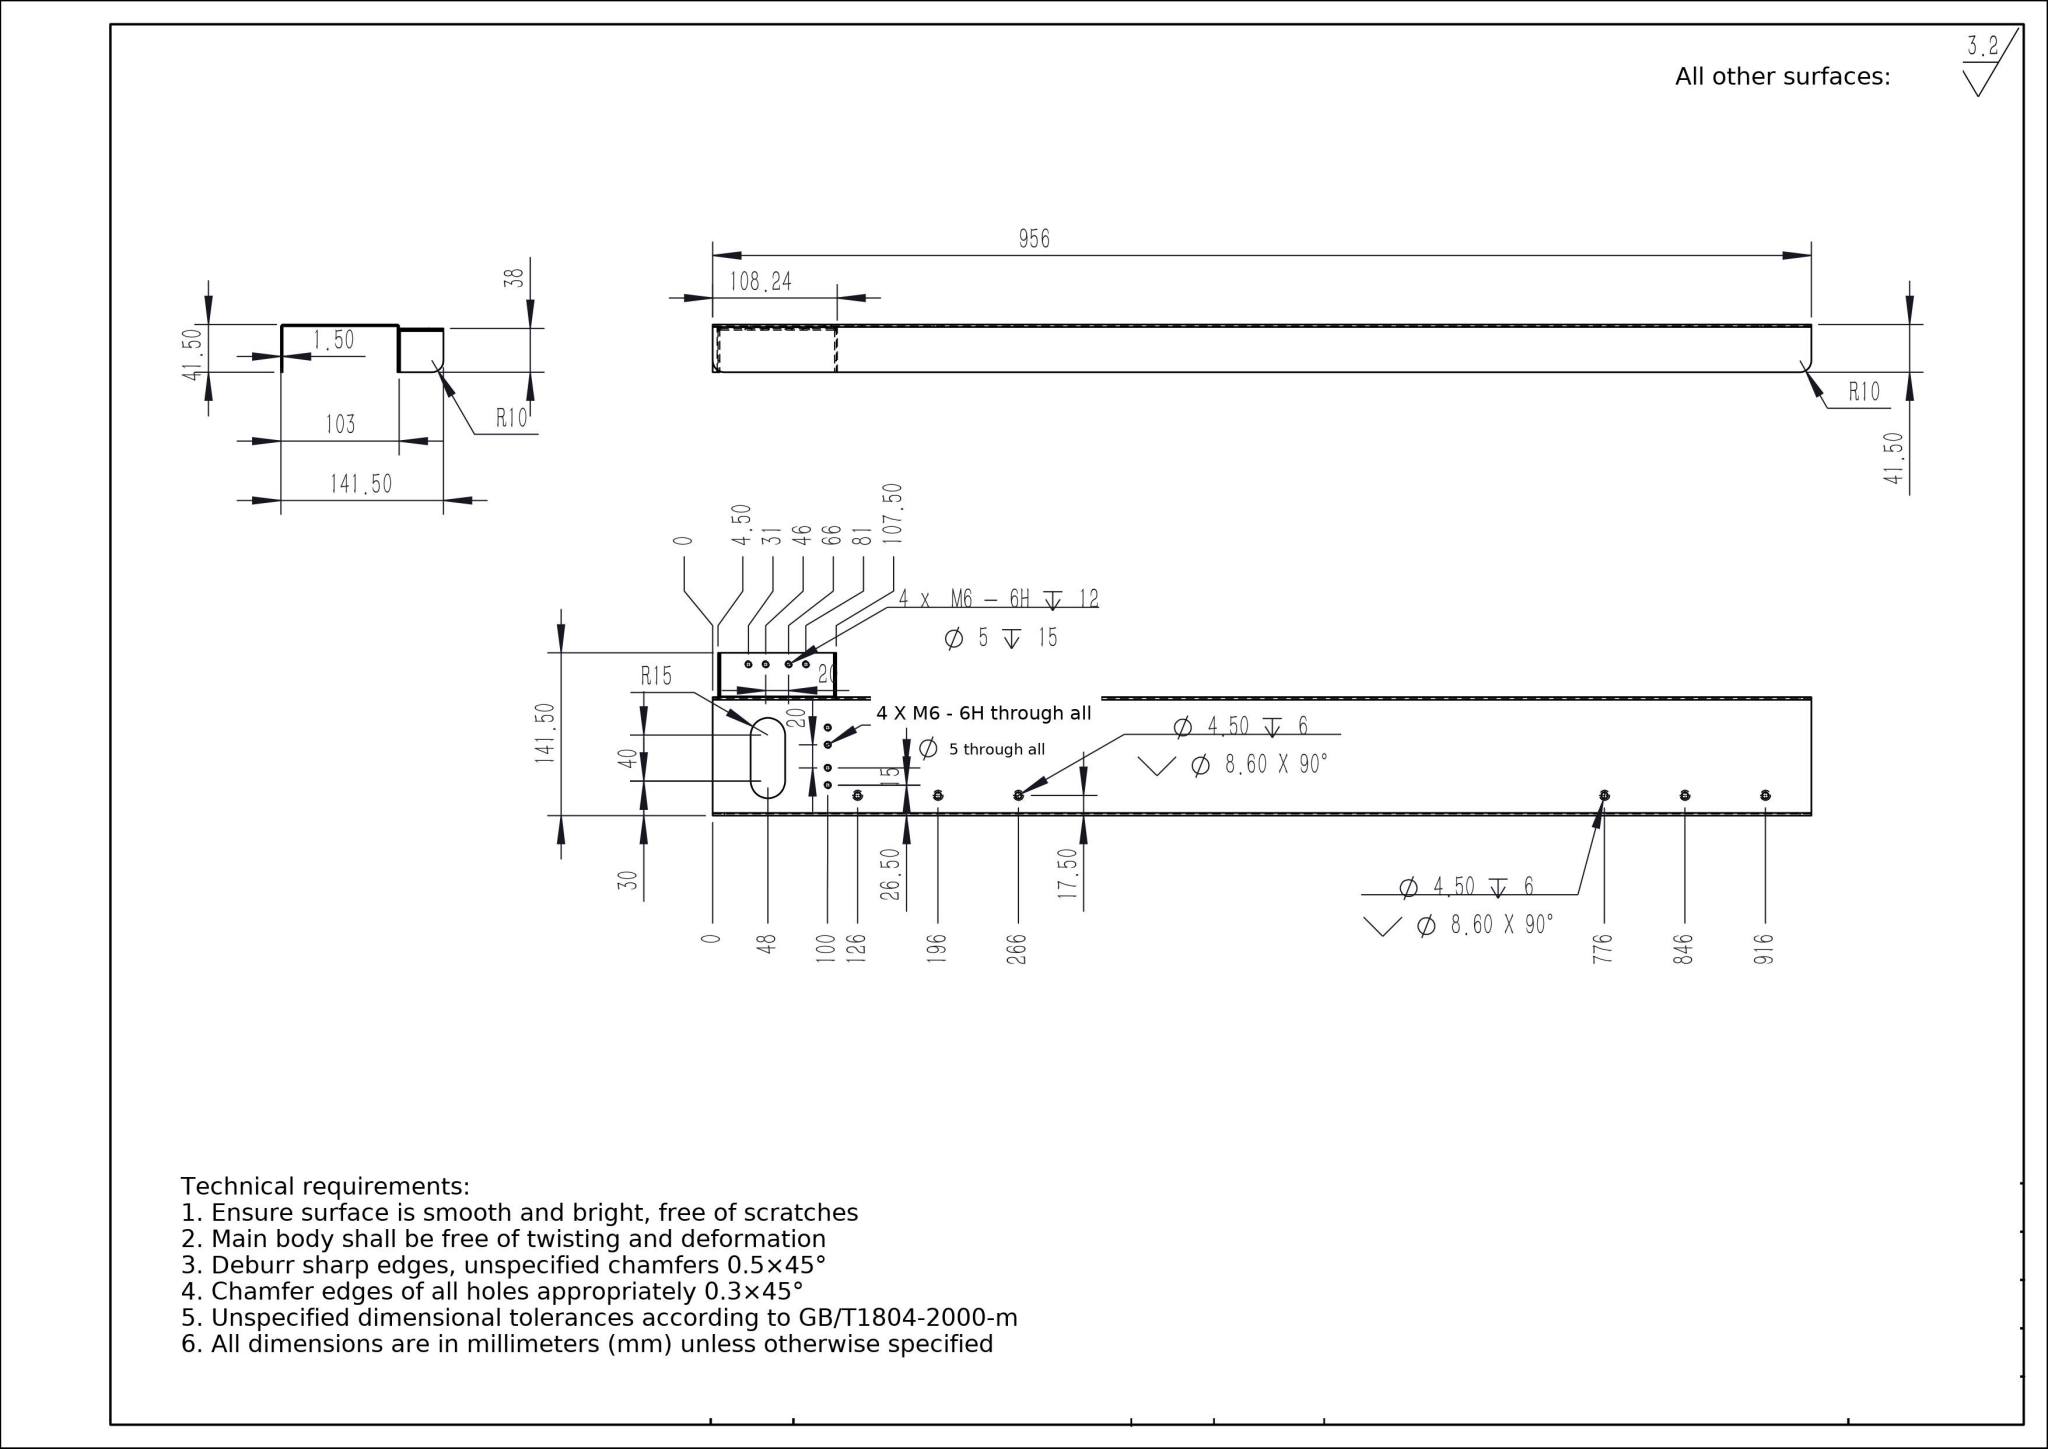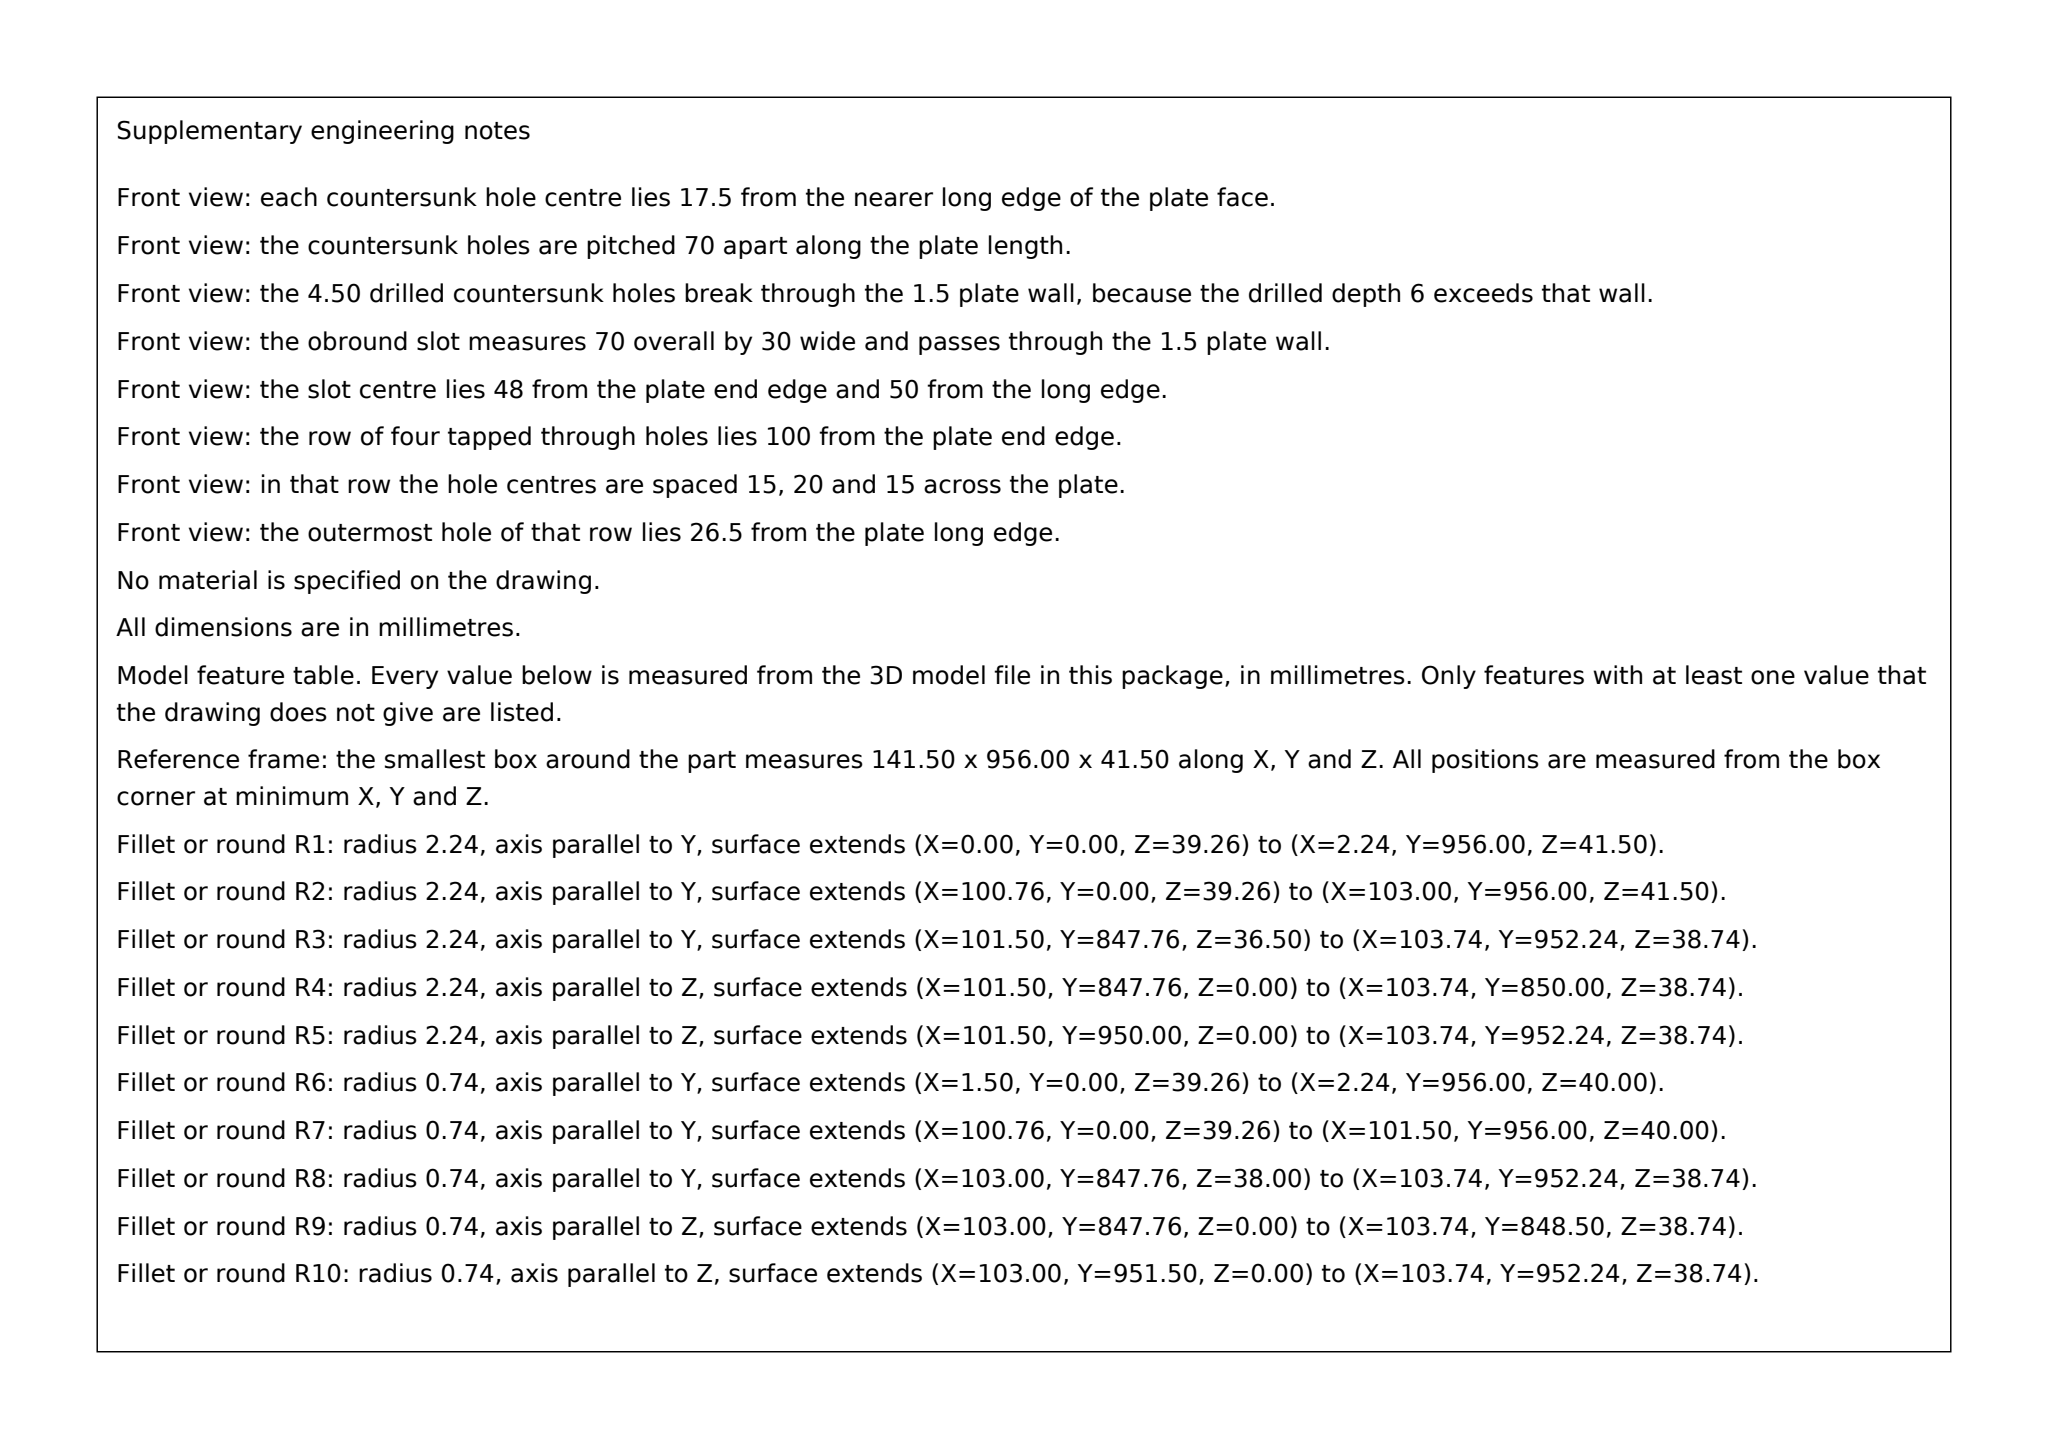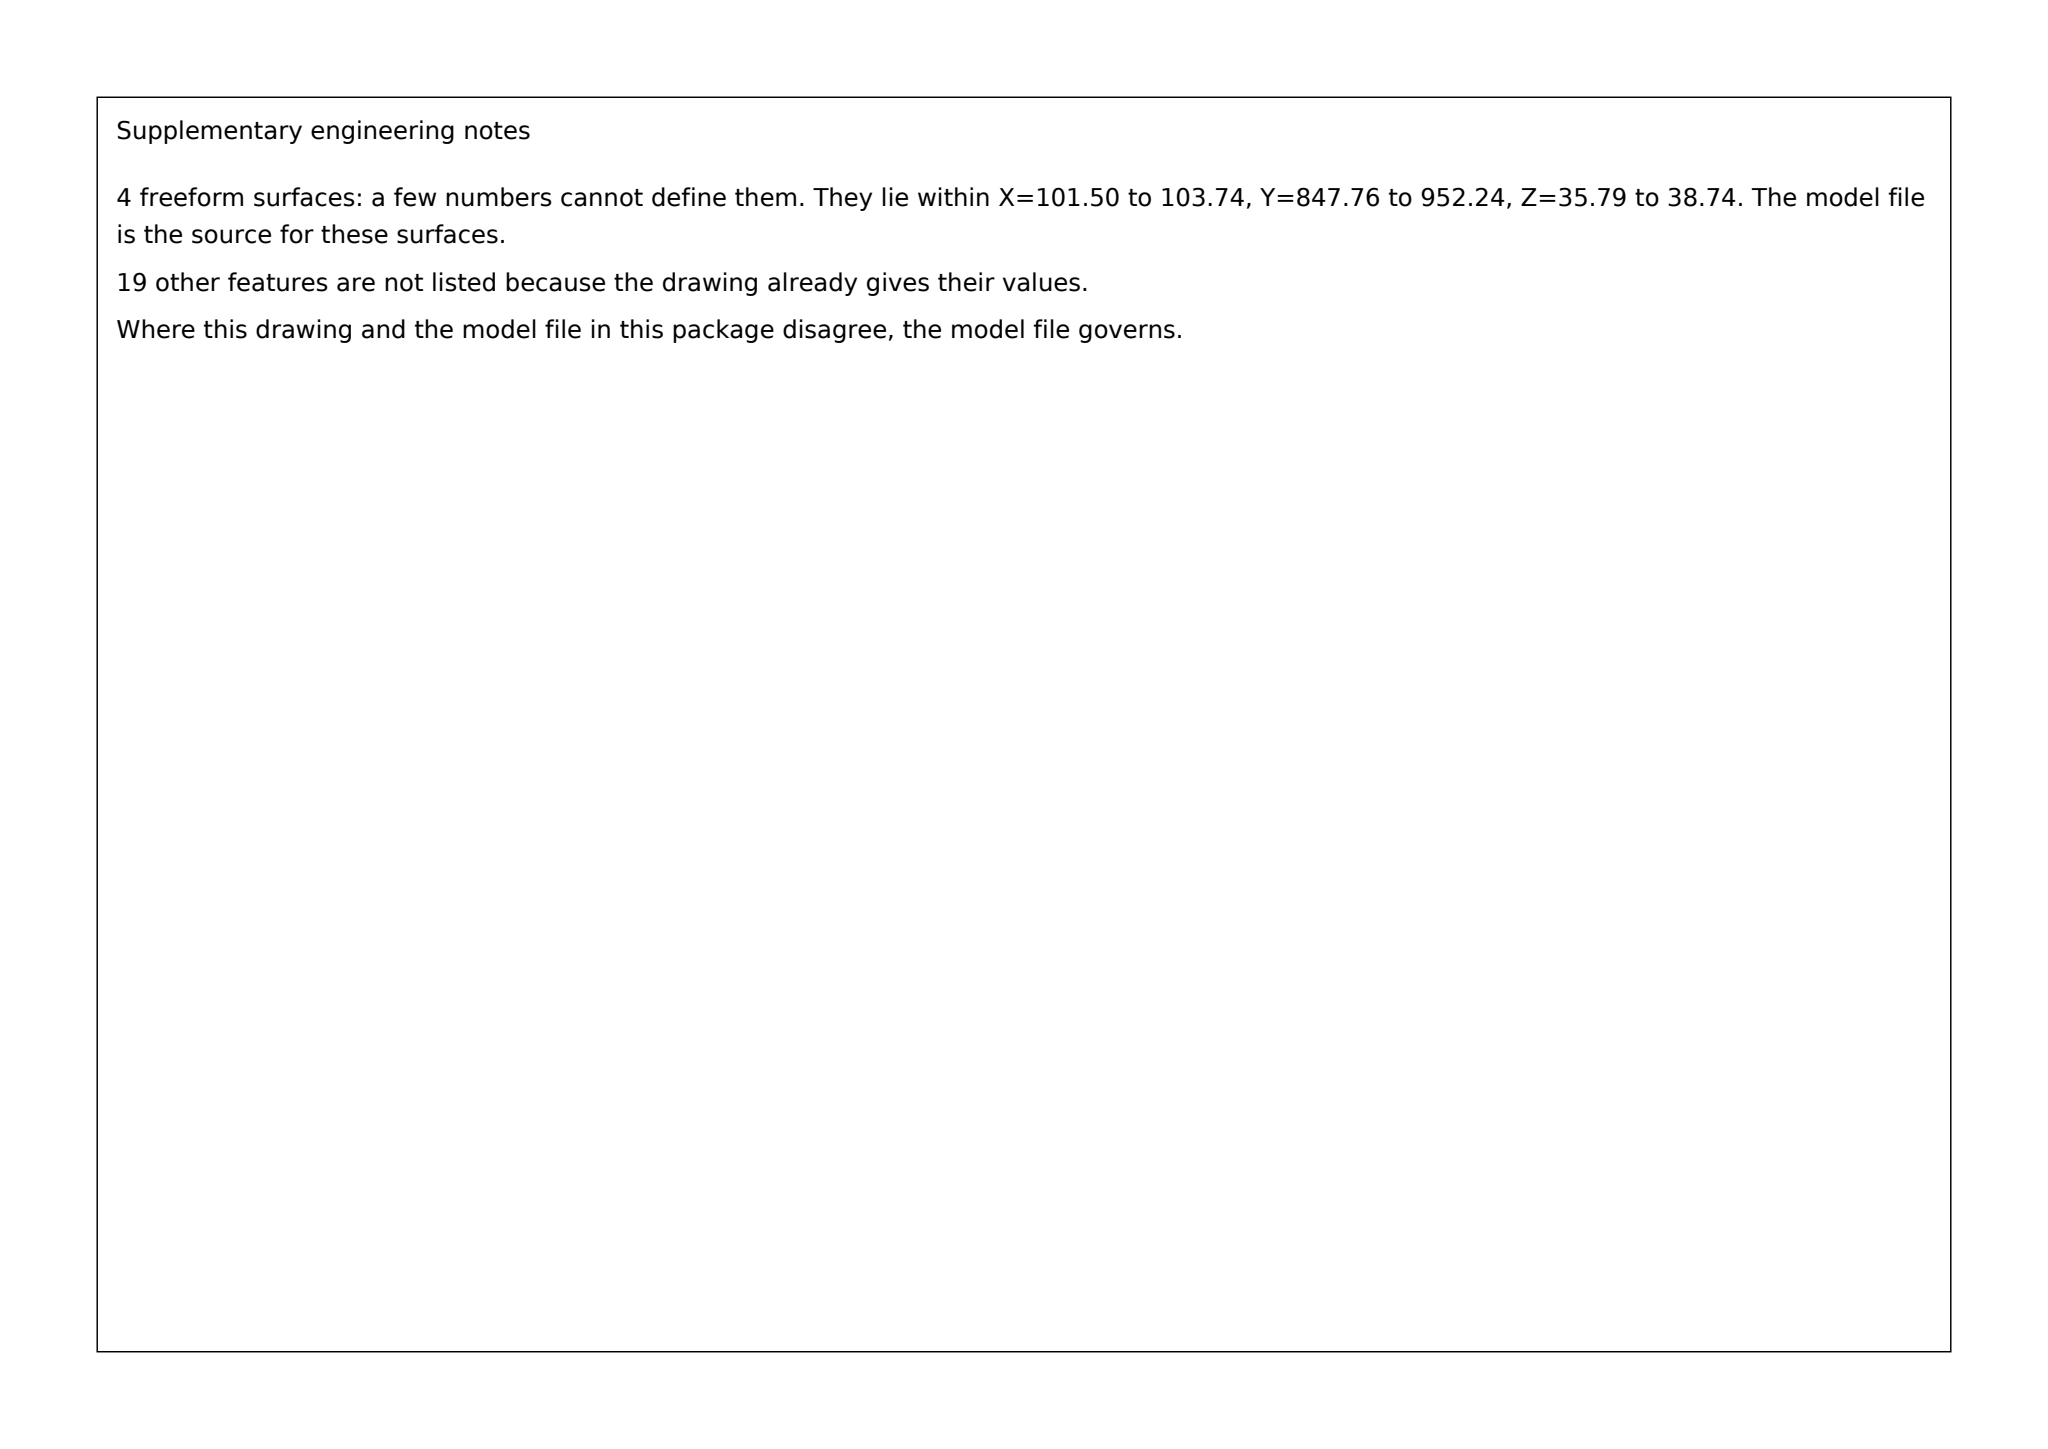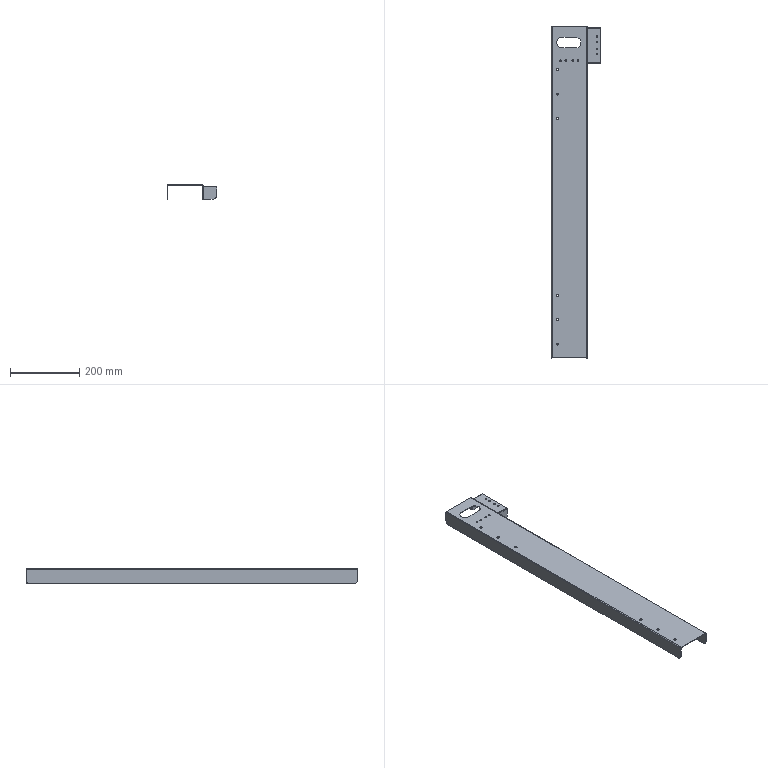Part | SolidWorks | mm | 1 solid | 88 faces | box 141.5 x 956 x 41.5 mm | volume 261159 mm3 | plane 38 | cylinder 34 | cone 12 | spline 4 | commonest cylinder face diameters 5 x16 1.473 x5 4.473 x5 20 x5 30 x3
Drawing notes:
R15 SLOT 30 WIDE X 70 LG, CTRS 30 & 70 FM EDGE, CL 48 FM END | from the solid: Ø30 z-axis cyls at (30,908) & (70,908), len 1.5; 956-908=48
FORMED CORNERS OF 1.50 WALL: OUTER R2.24, INNER R0.74, TYP | from the solid: Cyl dia 1.473 (R0.74 inner) & 4.473 (R2.24 outer), axis y at x=2.24/100.76 z=39.26 L956, and axis z at (103.74,847.76)/(103.74,952.24) L38.74
SIDE WALLS: 2X Ø20 THRU AT 10, 1X Ø20 THRU AT 946; CL 10 UP | from the solid: Ø20 arcs with axis along X at (y=10, z=10) occur twice - from x=0 to 1.5 and from x=101.5 to 103.0 (one in each 1.50 side wall), while only one Ø20 arc axis along X lies at (y=946, z=10) from x=0 to 1.5; all centre lines Z=10.00 above base
END WALLS: 2X Ø20 THRU, CL 131.50 ACROSS WIDTH, 10 UP FROM BASE | from the solid: Cyl dia20 axis y at x=131.5 z=10, L1.5, count 2 (both y=0 and y=956 end walls)
4X M6-6H THRU 1.50 END WALL (Ø5 THRU PILOT) ON CL X=131.50, i.e. 10.00 FROM THE 141.50 EDGE; HOLES AT 31, 46, 66, 81 FROM THE 956 END | from the solid: cylinders [5.0,"z",[131.5,875/890/910/925],1.5] with bbox_xyz X=141.5, Y=956
4X M6-6H THRU 1.50 WALL (Ø5 THRU) IN ROW 100 FROM THE 956 END: X = 26.50, 41.50, 61.50, 76.50 FROM X0 DATUM (SPACING 15 / 20 / 15) | from the solid: cylinders [5.0,"z",[26.5/41.5/61.5/76.5,856.0],1.5]
FORMED END BOX: TOP FACE 38.00 ABOVE BASE (Z0); 1.50 RAISED WALL PLANE AT X=103.00 FROM X0 | from the solid: axis_planes ["z",38.0] and ["x",103.0]